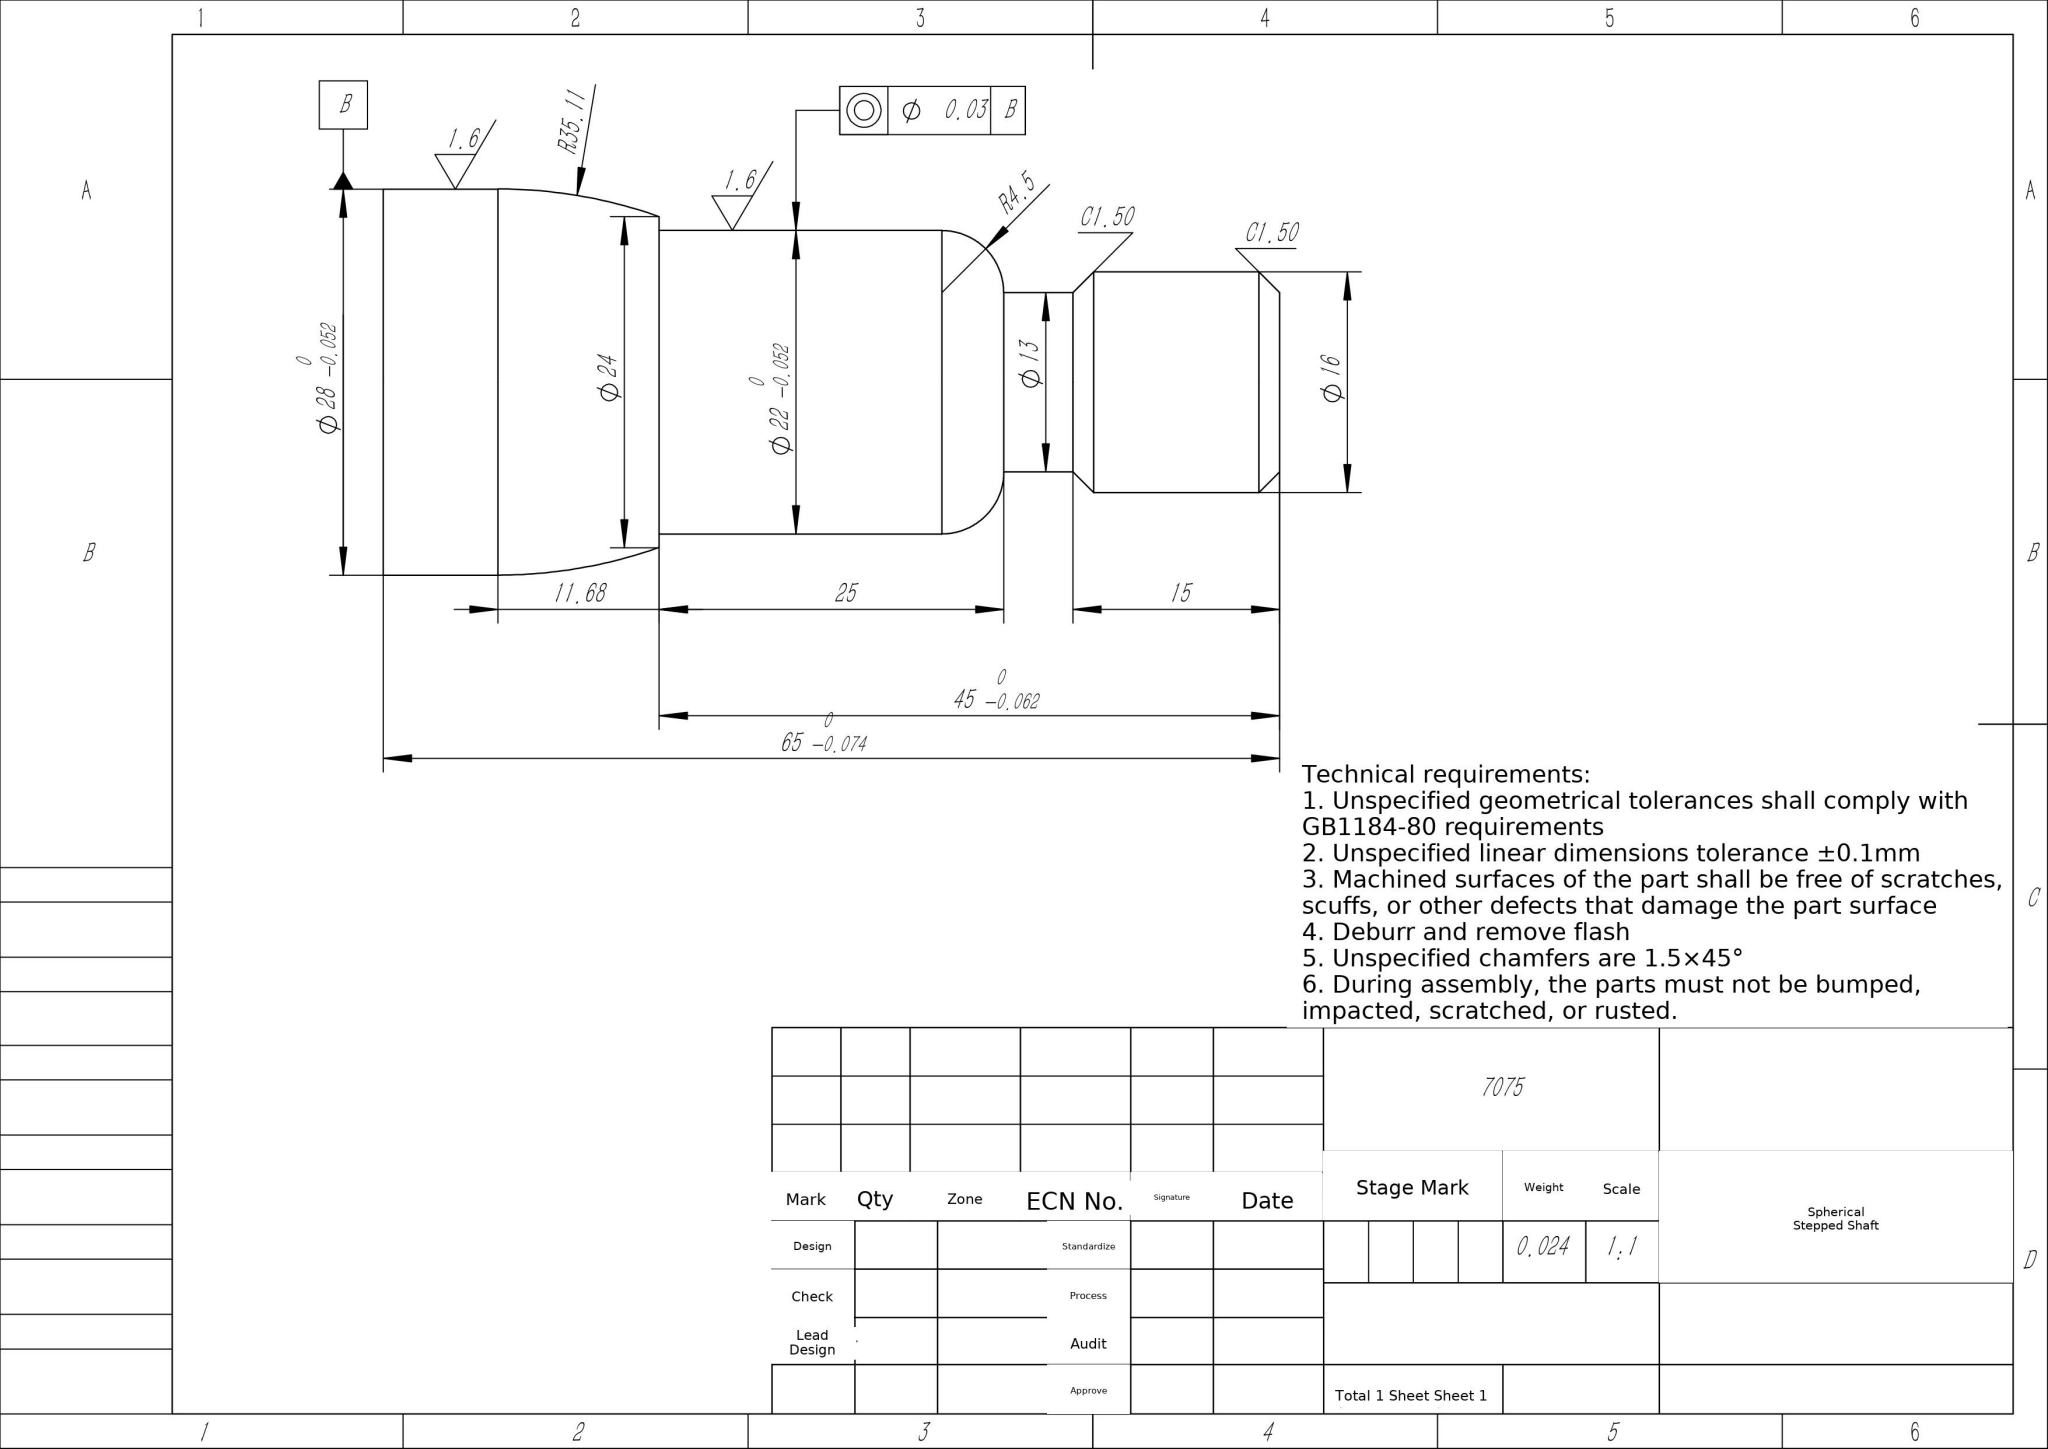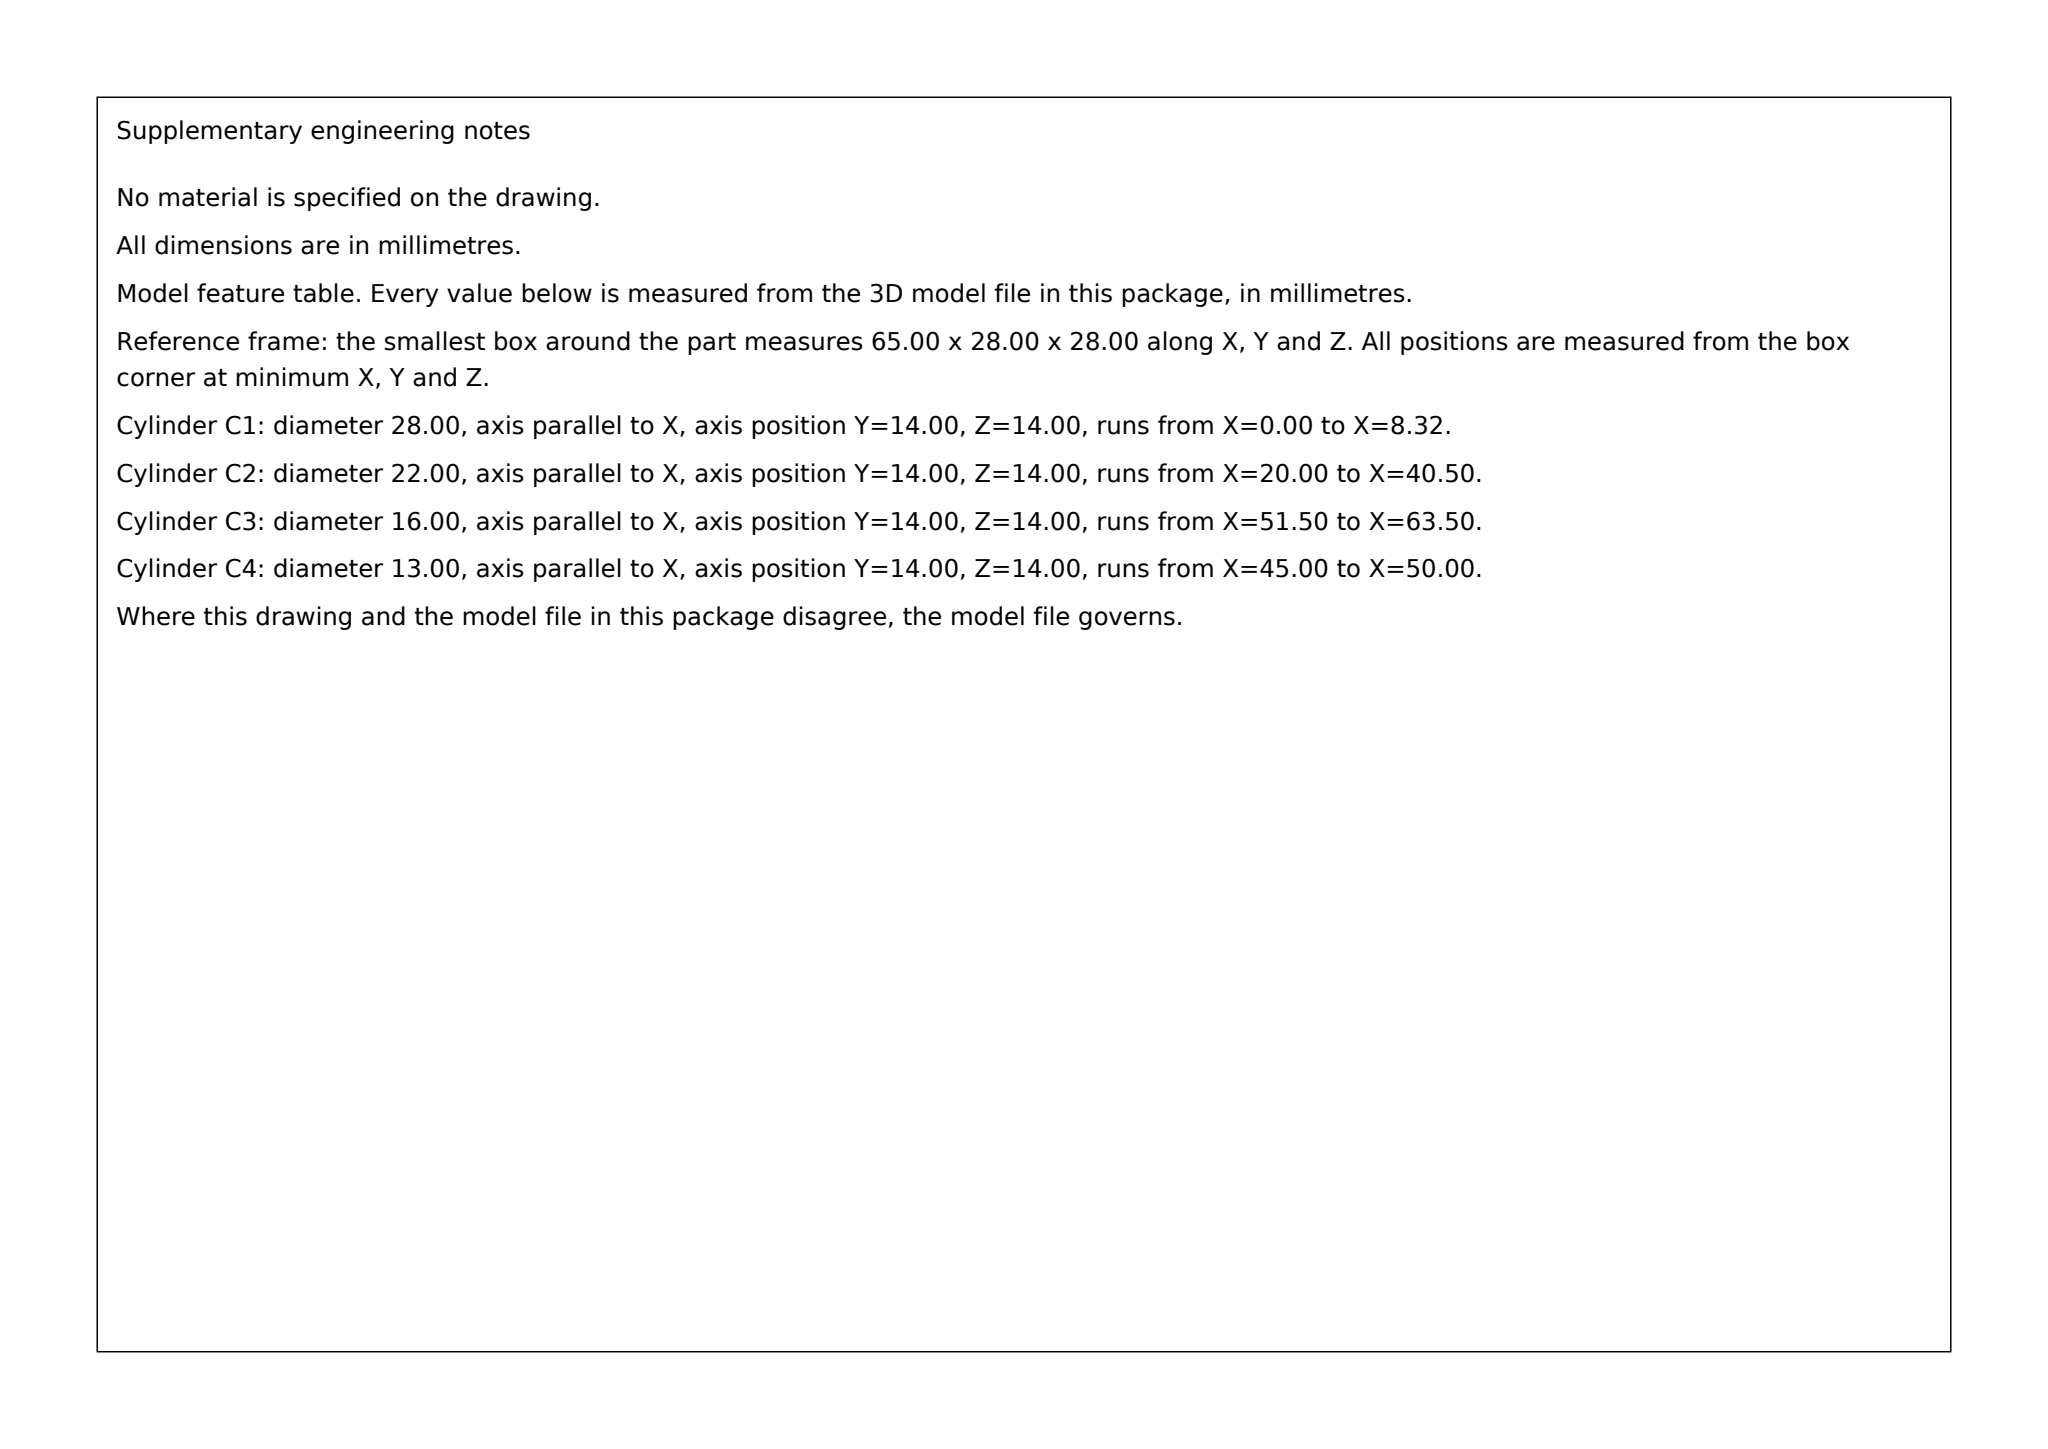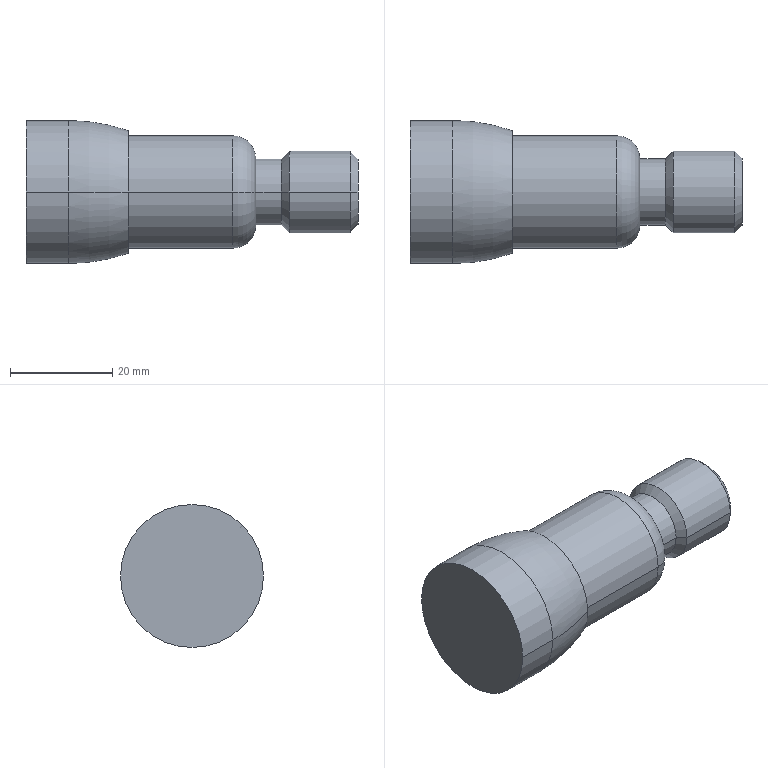Part | SolidWorks | mm | material 7075 | 1 solid | 19 faces | box 65 x 28 x 28 mm | volume 24471 mm3 | cylinder 8 | torus 4 | cone 4 | plane 3 | commonest cylinder face diameters 13 x2 16 x2 22 x2 28 x2
STEP:
#1=CARTESIAN_POINT('',(40.5,-11.,0.));
#2=VERTEX_POINT('',#1);
#3=CARTESIAN_POINT('',(40.5,11.,0.));
#4=VERTEX_POINT('',#3);
#5=CARTESIAN_POINT('',(40.5,0.,0.));
#6=DIRECTION('',(-1.,-0.,0.));
#7=DIRECTION('',(0.,1.,0.));
#8=AXIS2_PLACEMENT_3D('',#5,#6,#7);
#9=CIRCLE('',#8,11.);
#10=EDGE_CURVE('',#2,#4,#9,.T.);
#11=ORIENTED_EDGE('',*,*,#10,.F.);
#12=CARTESIAN_POINT('',(45.,-6.5,0.));
#13=VERTEX_POINT('',#12);
#14=CARTESIAN_POINT('',(40.5,-6.5,0.));
#15=DIRECTION('',(-0.,0.,1.));
#16=DIRECTION('',(0.,-1.,0.));
#17=AXIS2_PLACEMENT_3D('',#14,#15,#16);
#18=CIRCLE('',#17,4.5);
#19=EDGE_CURVE('',#2,#13,#18,.T.);
#20=ORIENTED_EDGE('',*,*,#19,.T.);
#21=CARTESIAN_POINT('',(45.,6.5,0.));
#22=VERTEX_POINT('',#21);
#23=CARTESIAN_POINT('',(45.,0.,0.));
#24=DIRECTION('',(1.,0.,0.));
#25=DIRECTION('',(0.,1.,0.));
#26=AXIS2_PLACEMENT_3D('',#23,#24,#25);
#27=CIRCLE('',#26,6.5);
#28=EDGE_CURVE('',#22,#13,#27,.T.);
#29=ORIENTED_EDGE('',*,*,#28,.F.);
#30=CARTESIAN_POINT('',(40.5,6.5,0.));
#31=DIRECTION('',(0.,0.,-1.));
#32=DIRECTION('',(-1.,0.,0.));
#33=AXIS2_PLACEMENT_3D('',#30,#31,#32);
#34=CIRCLE('',#33,4.5);
#35=EDGE_CURVE('',#4,#22,#34,.T.);
#36=ORIENTED_EDGE('',*,*,#35,.F.);
#37=EDGE_LOOP('',(#11,#20,#29,#36));
#38=FACE_OUTER_BOUND('',#37,.T.);
#39=CARTESIAN_POINT('',(40.5,0.,0.));
#40=DIRECTION('',(1.,0.,0.));
#41=DIRECTION('',(-0.,1.,0.));
#42=AXIS2_PLACEMENT_3D('',#39,#40,#41);
#43=TOROIDAL_SURFACE('',#42,6.5,4.5);
#44=ADVANCED_FACE('',(#38),#43,.T.);
#45=CARTESIAN_POINT('',(50.,6.5,0.));
#46=VERTEX_POINT('',#45);
#47=CARTESIAN_POINT('',(50.,-6.5,0.));
#48=VERTEX_POINT('',#47);
#49=CARTESIAN_POINT('',(50.,0.,0.));
#50=DIRECTION('',(1.,0.,0.));
#51=DIRECTION('',(0.,1.,0.));
#52=AXIS2_PLACEMENT_3D('',#49,#50,#51);
#53=CIRCLE('',#52,6.5);
#54=EDGE_CURVE('',#46,#48,#53,.T.);
#55=ORIENTED_EDGE('',*,*,#54,.T.);
#56=CARTESIAN_POINT('',(51.5,-8.,0.));
#57=VERTEX_POINT('',#56);
#58=CARTESIAN_POINT('',(51.5,-8.,0.));
#59=DIRECTION('',(0.7071,-0.7071,0.));
#60=VECTOR('',#59,1000.);
#61=LINE('',#58,#60);
#62=EDGE_CURVE('',#48,#57,#61,.T.);
#63=ORIENTED_EDGE('',*,*,#62,.T.);
#64=CARTESIAN_POINT('',(51.5,8.,0.));
#65=VERTEX_POINT('',#64);
#66=CARTESIAN_POINT('',(51.5,0.,0.));
#67=DIRECTION('',(1.,0.,0.));
#68=DIRECTION('',(0.,-1.,0.));
#69=AXIS2_PLACEMENT_3D('',#66,#67,#68);
#70=CIRCLE('',#69,8.);
#71=EDGE_CURVE('',#65,#57,#70,.T.);
#72=ORIENTED_EDGE('',*,*,#71,.F.);
#73=CARTESIAN_POINT('',(51.5,8.,0.));
#74=DIRECTION('',(0.7071,0.7071,0.));
#75=VECTOR('',#74,1000.);
#76=LINE('',#73,#75);
#77=EDGE_CURVE('',#46,#65,#76,.T.);
#78=ORIENTED_EDGE('',*,*,#77,.F.);
#79=EDGE_LOOP('',(#55,#63,#72,#78));
#80=FACE_OUTER_BOUND('',#79,.T.);
#81=CARTESIAN_POINT('',(51.5,0.,0.));
#82=DIRECTION('',(1.,0.,0.));
#83=DIRECTION('',(0.,1.,0.));
#84=AXIS2_PLACEMENT_3D('',#81,#82,#83);
#85=CONICAL_SURFACE('',#84,8.,0.7854);
#86=ADVANCED_FACE('',(#80),#85,.T.);
#87=CARTESIAN_POINT('',(65.,6.5,0.));
#88=VERTEX_POINT('',#87);
#89=CARTESIAN_POINT('',(65.,-6.5,0.));
#90=VERTEX_POINT('',#89);
#91=CARTESIAN_POINT('',(65.,0.,0.));
#92=DIRECTION('',(1.,0.,0.));
#93=DIRECTION('',(0.,1.,0.));
#94=AXIS2_PLACEMENT_3D('',#91,#92,#93);
#95=CIRCLE('',#94,6.5);
#96=EDGE_CURVE('',#88,#90,#95,.T.);
#97=ORIENTED_EDGE('',*,*,#96,.F.);
#98=CARTESIAN_POINT('',(63.5,8.,0.));
#99=VERTEX_POINT('',#98);
#100=CARTESIAN_POINT('',(65.,6.5,0.));
#101=DIRECTION('',(-0.7071,0.7071,0.));
#102=VECTOR('',#101,1000.);
#103=LINE('',#100,#102);
#104=EDGE_CURVE('',#88,#99,#103,.T.);
#105=ORIENTED_EDGE('',*,*,#104,.T.);
#106=CARTESIAN_POINT('',(63.5,-8.,0.));
#107=VERTEX_POINT('',#106);
#108=CARTESIAN_POINT('',(63.5,0.,0.));
#109=DIRECTION('',(-1.,-0.,0.));
#110=DIRECTION('',(0.,1.,0.));
#111=AXIS2_PLACEMENT_3D('',#108,#109,#110);
#112=CIRCLE('',#111,8.);
#113=EDGE_CURVE('',#107,#99,#112,.T.);
#114=ORIENTED_EDGE('',*,*,#113,.F.);
#115=CARTESIAN_POINT('',(65.,-6.5,0.));
#116=DIRECTION('',(-0.7071,-0.7071,0.));
#117=VECTOR('',#116,1000.);
#118=LINE('',#115,#117);
#119=EDGE_CURVE('',#90,#107,#118,.T.);
#120=ORIENTED_EDGE('',*,*,#119,.F.);
#121=EDGE_LOOP('',(#97,#105,#114,#120));
#122=FACE_OUTER_BOUND('',#121,.T.);
#123=CARTESIAN_POINT('',(65.,0.,0.));
#124=DIRECTION('',(-1.,-0.,0.));
#125=DIRECTION('',(0.,-1.,0.));
#126=AXIS2_PLACEMENT_3D('',#123,#124,#125);
#127=CONICAL_SURFACE('',#126,6.5,0.7854);
#128=ADVANCED_FACE('',(#122),#127,.T.);
#129=ORIENTED_EDGE('',*,*,#71,.T.);
#130=CARTESIAN_POINT('',(65.,-8.,0.));
#131=DIRECTION('',(1.,0.,0.));
#132=VECTOR('',#131,1000.);
#133=LINE('',#130,#132);
#134=EDGE_CURVE('',#57,#107,#133,.T.);
#135=ORIENTED_EDGE('',*,*,#134,.T.);
#136=ORIENTED_EDGE('',*,*,#113,.T.);
#137=CARTESIAN_POINT('',(65.,8.,0.));
#138=DIRECTION('',(1.,0.,0.));
#139=VECTOR('',#138,1000.);
#140=LINE('',#137,#139);
#141=EDGE_CURVE('',#65,#99,#140,.T.);
#142=ORIENTED_EDGE('',*,*,#141,.F.);
#143=EDGE_LOOP('',(#129,#135,#136,#142));
#144=FACE_OUTER_BOUND('',#143,.T.);
#145=CARTESIAN_POINT('',(65.,0.,0.));
#146=DIRECTION('',(1.,0.,0.));
#147=DIRECTION('',(0.,1.,0.));
#148=AXIS2_PLACEMENT_3D('',#145,#146,#147);
#149=CYLINDRICAL_SURFACE('',#148,8.);
#150=ADVANCED_FACE('',(#144),#149,.T.);
#151=ORIENTED_EDGE('',*,*,#28,.T.);
#152=CARTESIAN_POINT('',(65.,-6.5,0.));
#153=DIRECTION('',(1.,0.,0.));
#154=VECTOR('',#153,1000.);
#155=LINE('',#152,#154);
#156=EDGE_CURVE('',#13,#48,#155,.T.);
#157=ORIENTED_EDGE('',*,*,#156,.T.);
#158=ORIENTED_EDGE('',*,*,#54,.F.);
#159=CARTESIAN_POINT('',(65.,6.5,0.));
#160=DIRECTION('',(1.,0.,0.));
#161=VECTOR('',#160,1000.);
#162=LINE('',#159,#161);
#163=EDGE_CURVE('',#22,#46,#162,.T.);
#164=ORIENTED_EDGE('',*,*,#163,.F.);
#165=EDGE_LOOP('',(#151,#157,#158,#164));
#166=FACE_OUTER_BOUND('',#165,.T.);
#167=CARTESIAN_POINT('',(65.,0.,0.));
#168=DIRECTION('',(1.,0.,0.));
#169=DIRECTION('',(0.,1.,0.));
#170=AXIS2_PLACEMENT_3D('',#167,#168,#169);
#171=CYLINDRICAL_SURFACE('',#170,6.5);
#172=ADVANCED_FACE('',(#166),#171,.T.);
#173=CARTESIAN_POINT('',(20.,11.,0.));
#174=VERTEX_POINT('',#173);
#175=CARTESIAN_POINT('',(20.,-11.,0.));
#176=VERTEX_POINT('',#175);
#177=CARTESIAN_POINT('',(20.,0.,0.));
#178=DIRECTION('',(1.,0.,0.));
#179=DIRECTION('',(0.,1.,0.));
#180=AXIS2_PLACEMENT_3D('',#177,#178,#179);
#181=CIRCLE('',#180,11.);
#182=EDGE_CURVE('',#174,#176,#181,.T.);
#183=ORIENTED_EDGE('',*,*,#182,.T.);
#184=CARTESIAN_POINT('',(65.,-11.,0.));
#185=DIRECTION('',(1.,0.,0.));
#186=VECTOR('',#185,1000.);
#187=LINE('',#184,#186);
#188=EDGE_CURVE('',#176,#2,#187,.T.);
#189=ORIENTED_EDGE('',*,*,#188,.T.);
#190=ORIENTED_EDGE('',*,*,#10,.T.);
#191=CARTESIAN_POINT('',(65.,11.,0.));
#192=DIRECTION('',(1.,0.,0.));
#193=VECTOR('',#192,1000.);
#194=LINE('',#191,#193);
#195=EDGE_CURVE('',#174,#4,#194,.T.);
#196=ORIENTED_EDGE('',*,*,#195,.F.);
#197=EDGE_LOOP('',(#183,#189,#190,#196));
#198=FACE_OUTER_BOUND('',#197,.T.);
#199=CARTESIAN_POINT('',(65.,0.,0.));
#200=DIRECTION('',(1.,0.,0.));
#201=DIRECTION('',(0.,1.,0.));
#202=AXIS2_PLACEMENT_3D('',#199,#200,#201);
#203=CYLINDRICAL_SURFACE('',#202,11.);
#204=ADVANCED_FACE('',(#198),#203,.T.);
#205=CARTESIAN_POINT('',(8.32,14.,0.));
#206=VERTEX_POINT('',#205);
#207=CARTESIAN_POINT('',(8.32,-14.,0.));
#208=VERTEX_POINT('',#207);
#209=CARTESIAN_POINT('',(8.32,0.,0.));
#210=DIRECTION('',(1.,0.,0.));
#211=DIRECTION('',(0.,1.,0.));
#212=AXIS2_PLACEMENT_3D('',#209,#210,#211);
#213=CIRCLE('',#212,14.);
#214=EDGE_CURVE('',#206,#208,#213,.T.);
#215=ORIENTED_EDGE('',*,*,#214,.T.);
#216=CARTESIAN_POINT('',(20.,-12.,0.));
#217=VERTEX_POINT('',#216);
#218=CARTESIAN_POINT('',(8.32,21.108,-0.));
#219=DIRECTION('',(-0.,0.,1.));
#220=DIRECTION('',(0.,-1.,0.));
#221=AXIS2_PLACEMENT_3D('',#218,#219,#220);
#222=CIRCLE('',#221,35.108);
#223=EDGE_CURVE('',#208,#217,#222,.T.);
#224=ORIENTED_EDGE('',*,*,#223,.T.);
#225=CARTESIAN_POINT('',(20.,12.,0.));
#226=VERTEX_POINT('',#225);
#227=CARTESIAN_POINT('',(20.,0.,0.));
#228=DIRECTION('',(1.,0.,0.));
#229=DIRECTION('',(0.,1.,0.));
#230=AXIS2_PLACEMENT_3D('',#227,#228,#229);
#231=CIRCLE('',#230,12.);
#232=EDGE_CURVE('',#226,#217,#231,.T.);
#233=ORIENTED_EDGE('',*,*,#232,.F.);
#234=CARTESIAN_POINT('',(8.32,-21.108,0.));
#235=DIRECTION('',(0.,0.,-1.));
#236=DIRECTION('',(-1.,0.,0.));
#237=AXIS2_PLACEMENT_3D('',#234,#235,#236);
#238=CIRCLE('',#237,35.108);
#239=EDGE_CURVE('',#206,#226,#238,.T.);
#240=ORIENTED_EDGE('',*,*,#239,.F.);
#241=EDGE_LOOP('',(#215,#224,#233,#240));
#242=FACE_OUTER_BOUND('',#241,.T.);
#243=CARTESIAN_POINT('',(8.32,0.,0.));
#244=DIRECTION('',(1.,0.,0.));
#245=DIRECTION('',(-0.,1.,0.));
#246=AXIS2_PLACEMENT_3D('',#243,#244,#245);
#247=TOROIDAL_SURFACE('',#246,-21.108,35.108);
#248=ADVANCED_FACE('',(#242),#247,.T.);
#249=CARTESIAN_POINT('',(-0.,14.,0.));
#250=VERTEX_POINT('',#249);
#251=CARTESIAN_POINT('',(0.,-14.,0.));
#252=VERTEX_POINT('',#251);
#253=CARTESIAN_POINT('',(0.,0.,0.));
#254=DIRECTION('',(1.,0.,0.));
#255=DIRECTION('',(-0.,1.,0.));
#256=AXIS2_PLACEMENT_3D('',#253,#254,#255);
#257=CIRCLE('',#256,14.);
#258=EDGE_CURVE('',#250,#252,#257,.T.);
#259=ORIENTED_EDGE('',*,*,#258,.T.);
#260=CARTESIAN_POINT('',(65.,-14.,0.));
#261=DIRECTION('',(1.,0.,0.));
#262=VECTOR('',#261,1000.);
#263=LINE('',#260,#262);
#264=EDGE_CURVE('',#252,#208,#263,.T.);
#265=ORIENTED_EDGE('',*,*,#264,.T.);
#266=ORIENTED_EDGE('',*,*,#214,.F.);
#267=CARTESIAN_POINT('',(65.,14.,0.));
#268=DIRECTION('',(1.,0.,0.));
#269=VECTOR('',#268,1000.);
#270=LINE('',#267,#269);
#271=EDGE_CURVE('',#250,#206,#270,.T.);
#272=ORIENTED_EDGE('',*,*,#271,.F.);
#273=EDGE_LOOP('',(#259,#265,#266,#272));
#274=FACE_OUTER_BOUND('',#273,.T.);
#275=CARTESIAN_POINT('',(65.,0.,0.));
#276=DIRECTION('',(1.,0.,0.));
#277=DIRECTION('',(0.,1.,0.));
#278=AXIS2_PLACEMENT_3D('',#275,#276,#277);
#279=CYLINDRICAL_SURFACE('',#278,14.);
#280=ADVANCED_FACE('',(#274),#279,.T.);
#281=ORIENTED_EDGE('',*,*,#258,.F.);
#282=CARTESIAN_POINT('',(0.,0.,0.));
#283=DIRECTION('',(1.,0.,0.));
#284=DIRECTION('',(-0.,1.,0.));
#285=AXIS2_PLACEMENT_3D('',#282,#283,#284);
#286=CIRCLE('',#285,14.);
#287=EDGE_CURVE('',#252,#250,#286,.T.);
#288=ORIENTED_EDGE('',*,*,#287,.F.);
#289=EDGE_LOOP('',(#281,#288));
#290=FACE_OUTER_BOUND('',#289,.T.);
#291=CARTESIAN_POINT('',(0.,0.,0.));
#292=DIRECTION('',(-1.,-0.,0.));
#293=DIRECTION('',(0.,-1.,0.));
#294=AXIS2_PLACEMENT_3D('',#291,#292,#293);
#295=PLANE('',#294);
#296=ADVANCED_FACE('',(#290),#295,.T.);
#297=ORIENTED_EDGE('',*,*,#264,.F.);
#298=ORIENTED_EDGE('',*,*,#287,.T.);
#299=ORIENTED_EDGE('',*,*,#271,.T.);
#300=CARTESIAN_POINT('',(8.32,0.,0.));
#301=DIRECTION('',(1.,0.,0.));
#302=DIRECTION('',(0.,1.,0.));
#303=AXIS2_PLACEMENT_3D('',#300,#301,#302);
#304=CIRCLE('',#303,14.);
#305=EDGE_CURVE('',#208,#206,#304,.T.);
#306=ORIENTED_EDGE('',*,*,#305,.F.);
#307=EDGE_LOOP('',(#297,#298,#299,#306));
#308=FACE_OUTER_BOUND('',#307,.T.);
#309=CARTESIAN_POINT('',(65.,0.,0.));
#310=DIRECTION('',(1.,0.,0.));
#311=DIRECTION('',(0.,1.,0.));
#312=AXIS2_PLACEMENT_3D('',#309,#310,#311);
#313=CYLINDRICAL_SURFACE('',#312,14.);
#314=ADVANCED_FACE('',(#308),#313,.T.);
#315=ORIENTED_EDGE('',*,*,#223,.F.);
#316=ORIENTED_EDGE('',*,*,#305,.T.);
#317=ORIENTED_EDGE('',*,*,#239,.T.);
#318=CARTESIAN_POINT('',(20.,0.,0.));
#319=DIRECTION('',(1.,0.,0.));
#320=DIRECTION('',(0.,1.,0.));
#321=AXIS2_PLACEMENT_3D('',#318,#319,#320);
#322=CIRCLE('',#321,12.);
#323=EDGE_CURVE('',#217,#226,#322,.T.);
#324=ORIENTED_EDGE('',*,*,#323,.F.);
#325=EDGE_LOOP('',(#315,#316,#317,#324));
#326=FACE_OUTER_BOUND('',#325,.T.);
#327=CARTESIAN_POINT('',(8.32,0.,0.));
#328=DIRECTION('',(1.,0.,0.));
#329=DIRECTION('',(-0.,1.,0.));
#330=AXIS2_PLACEMENT_3D('',#327,#328,#329);
#331=TOROIDAL_SURFACE('',#330,-21.108,35.108);
#332=ADVANCED_FACE('',(#326),#331,.T.);
#333=ORIENTED_EDGE('',*,*,#232,.T.);
#334=ORIENTED_EDGE('',*,*,#323,.T.);
#335=EDGE_LOOP('',(#333,#334));
#336=FACE_OUTER_BOUND('',#335,.T.);
#337=ORIENTED_EDGE('',*,*,#182,.F.);
#338=CARTESIAN_POINT('',(20.,0.,0.));
#339=DIRECTION('',(1.,0.,0.));
#340=DIRECTION('',(0.,1.,0.));
#341=AXIS2_PLACEMENT_3D('',#338,#339,#340);
#342=CIRCLE('',#341,11.);
#343=EDGE_CURVE('',#176,#174,#342,.T.);
#344=ORIENTED_EDGE('',*,*,#343,.F.);
#345=EDGE_LOOP('',(#337,#344));
#346=FACE_BOUND('',#345,.T.);
#347=CARTESIAN_POINT('',(20.,12.,0.));
#348=DIRECTION('',(1.,0.,0.));
#349=DIRECTION('',(-0.,1.,0.));
#350=AXIS2_PLACEMENT_3D('',#347,#348,#349);
#351=PLANE('',#350);
#352=ADVANCED_FACE('',(#336,#346),#351,.T.);
#353=ORIENTED_EDGE('',*,*,#188,.F.);
#354=ORIENTED_EDGE('',*,*,#343,.T.);
#355=ORIENTED_EDGE('',*,*,#195,.T.);
#356=CARTESIAN_POINT('',(40.5,0.,0.));
#357=DIRECTION('',(-1.,-0.,0.));
#358=DIRECTION('',(0.,1.,0.));
#359=AXIS2_PLACEMENT_3D('',#356,#357,#358);
#360=CIRCLE('',#359,11.);
#361=EDGE_CURVE('',#4,#2,#360,.T.);
#362=ORIENTED_EDGE('',*,*,#361,.T.);
#363=EDGE_LOOP('',(#353,#354,#355,#362));
#364=FACE_OUTER_BOUND('',#363,.T.);
#365=CARTESIAN_POINT('',(65.,0.,0.));
#366=DIRECTION('',(1.,0.,0.));
#367=DIRECTION('',(0.,1.,0.));
#368=AXIS2_PLACEMENT_3D('',#365,#366,#367);
#369=CYLINDRICAL_SURFACE('',#368,11.);
#370=ADVANCED_FACE('',(#364),#369,.T.);
#371=ORIENTED_EDGE('',*,*,#156,.F.);
#372=CARTESIAN_POINT('',(45.,0.,0.));
#373=DIRECTION('',(1.,0.,0.));
#374=DIRECTION('',(0.,1.,0.));
#375=AXIS2_PLACEMENT_3D('',#372,#373,#374);
#376=CIRCLE('',#375,6.5);
#377=EDGE_CURVE('',#13,#22,#376,.T.);
#378=ORIENTED_EDGE('',*,*,#377,.T.);
#379=ORIENTED_EDGE('',*,*,#163,.T.);
#380=CARTESIAN_POINT('',(50.,0.,0.));
#381=DIRECTION('',(1.,0.,0.));
#382=DIRECTION('',(0.,1.,0.));
#383=AXIS2_PLACEMENT_3D('',#380,#381,#382);
#384=CIRCLE('',#383,6.5);
#385=EDGE_CURVE('',#48,#46,#384,.T.);
#386=ORIENTED_EDGE('',*,*,#385,.F.);
#387=EDGE_LOOP('',(#371,#378,#379,#386));
#388=FACE_OUTER_BOUND('',#387,.T.);
#389=CARTESIAN_POINT('',(65.,0.,0.));
#390=DIRECTION('',(1.,0.,0.));
#391=DIRECTION('',(0.,1.,0.));
#392=AXIS2_PLACEMENT_3D('',#389,#390,#391);
#393=CYLINDRICAL_SURFACE('',#392,6.5);
#394=ADVANCED_FACE('',(#388),#393,.T.);
#395=ORIENTED_EDGE('',*,*,#134,.F.);
#396=CARTESIAN_POINT('',(51.5,0.,0.));
#397=DIRECTION('',(1.,0.,0.));
#398=DIRECTION('',(0.,-1.,0.));
#399=AXIS2_PLACEMENT_3D('',#396,#397,#398);
#400=CIRCLE('',#399,8.);
#401=EDGE_CURVE('',#57,#65,#400,.T.);
#402=ORIENTED_EDGE('',*,*,#401,.T.);
#403=ORIENTED_EDGE('',*,*,#141,.T.);
#404=CARTESIAN_POINT('',(63.5,0.,0.));
#405=DIRECTION('',(-1.,-0.,0.));
#406=DIRECTION('',(0.,1.,0.));
#407=AXIS2_PLACEMENT_3D('',#404,#405,#406);
#408=CIRCLE('',#407,8.);
#409=EDGE_CURVE('',#99,#107,#408,.T.);
#410=ORIENTED_EDGE('',*,*,#409,.T.);
#411=EDGE_LOOP('',(#395,#402,#403,#410));
#412=FACE_OUTER_BOUND('',#411,.T.);
#413=CARTESIAN_POINT('',(65.,0.,0.));
#414=DIRECTION('',(1.,0.,0.));
#415=DIRECTION('',(0.,1.,0.));
#416=AXIS2_PLACEMENT_3D('',#413,#414,#415);
#417=CYLINDRICAL_SURFACE('',#416,8.);
#418=ADVANCED_FACE('',(#412),#417,.T.);
#419=CARTESIAN_POINT('',(65.,0.,0.));
#420=DIRECTION('',(1.,0.,0.));
#421=DIRECTION('',(0.,1.,0.));
#422=AXIS2_PLACEMENT_3D('',#419,#420,#421);
#423=CIRCLE('',#422,6.5);
#424=EDGE_CURVE('',#90,#88,#423,.T.);
#425=ORIENTED_EDGE('',*,*,#424,.T.);
#426=ORIENTED_EDGE('',*,*,#96,.T.);
#427=EDGE_LOOP('',(#425,#426));
#428=FACE_OUTER_BOUND('',#427,.T.);
#429=CARTESIAN_POINT('',(65.,8.,0.));
#430=DIRECTION('',(1.,0.,0.));
#431=DIRECTION('',(-0.,1.,0.));
#432=AXIS2_PLACEMENT_3D('',#429,#430,#431);
#433=PLANE('',#432);
#434=ADVANCED_FACE('',(#428),#433,.T.);
#435=ORIENTED_EDGE('',*,*,#104,.F.);
#436=ORIENTED_EDGE('',*,*,#424,.F.);
#437=ORIENTED_EDGE('',*,*,#119,.T.);
#438=ORIENTED_EDGE('',*,*,#409,.F.);
#439=EDGE_LOOP('',(#435,#436,#437,#438));
#440=FACE_OUTER_BOUND('',#439,.T.);
#441=CARTESIAN_POINT('',(65.,0.,0.));
#442=DIRECTION('',(-1.,-0.,0.));
#443=DIRECTION('',(0.,-1.,0.));
#444=AXIS2_PLACEMENT_3D('',#441,#442,#443);
#445=CONICAL_SURFACE('',#444,6.5,0.7854);
#446=ADVANCED_FACE('',(#440),#445,.T.);
#447=ORIENTED_EDGE('',*,*,#62,.F.);
#448=ORIENTED_EDGE('',*,*,#385,.T.);
#449=ORIENTED_EDGE('',*,*,#77,.T.);
#450=ORIENTED_EDGE('',*,*,#401,.F.);
#451=EDGE_LOOP('',(#447,#448,#449,#450));
#452=FACE_OUTER_BOUND('',#451,.T.);
#453=CARTESIAN_POINT('',(51.5,0.,0.));
#454=DIRECTION('',(1.,0.,0.));
#455=DIRECTION('',(0.,1.,0.));
#456=AXIS2_PLACEMENT_3D('',#453,#454,#455);
#457=CONICAL_SURFACE('',#456,8.,0.7854);
#458=ADVANCED_FACE('',(#452),#457,.T.);
#459=ORIENTED_EDGE('',*,*,#19,.F.);
#460=ORIENTED_EDGE('',*,*,#361,.F.);
#461=ORIENTED_EDGE('',*,*,#35,.T.);
#462=ORIENTED_EDGE('',*,*,#377,.F.);
#463=EDGE_LOOP('',(#459,#460,#461,#462));
#464=FACE_OUTER_BOUND('',#463,.T.);
#465=CARTESIAN_POINT('',(40.5,0.,0.));
#466=DIRECTION('',(1.,0.,0.));
#467=DIRECTION('',(-0.,1.,0.));
#468=AXIS2_PLACEMENT_3D('',#465,#466,#467);
#469=TOROIDAL_SURFACE('',#468,6.5,4.5);
#470=ADVANCED_FACE('',(#464),#469,.T.);
#471=CLOSED_SHELL('',(#44,#86,#128,#150,#172,#204,#248,#280,#296,#314,#332,#352,#370,#394,#418,#434,#446,#458,#470));
#472=MANIFOLD_SOLID_BREP('',#471);
#473=CARTESIAN_POINT('',(0.,0.,0.));
#474=DIRECTION('',(0.,0.,1.));
#475=DIRECTION('',(1.,0.,0.));
#476=AXIS2_PLACEMENT_3D('',#473,#474,#475);
#477=(LENGTH_UNIT()NAMED_UNIT(*)SI_UNIT(.MILLI.,.METRE.));
#478=UNCERTAINTY_MEASURE_WITH_UNIT(LENGTH_MEASURE(0.00001),#477,'','');
#479=(NAMED_UNIT(*)PLANE_ANGLE_UNIT()SI_UNIT($,.RADIAN.));
#480=(NAMED_UNIT(*)SI_UNIT($,.STERADIAN.)SOLID_ANGLE_UNIT());
#481=(GEOMETRIC_REPRESENTATION_CONTEXT(3)GLOBAL_UNCERTAINTY_ASSIGNED_CONTEXT((#478))GLOBAL_UNIT_ASSIGNED_CONTEXT((#477,#479,#480))REPRESENTATION_CONTEXT('',''));
#482=ADVANCED_BREP_SHAPE_REPRESENTATION('',(#472,#476),#481);